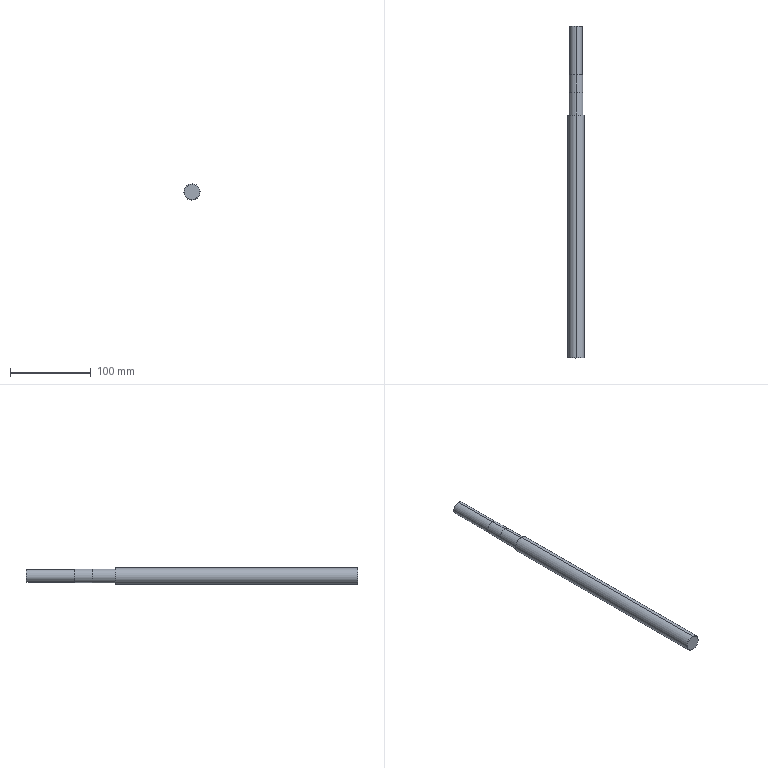Component | SolidWorks | ScrewRod-1 | 1 solid | 29 faces | box 20 x 410 x 20 mm | volume 116845 mm3 | cylinder 13 | cone 8 | plane 8 | commonest cylinder face diameters 5 x5 16 x2 16.7 x2 17 x2 20 x2
build123d program:
from build123d import *

# Parameters (mm, degrees)
SKETCH2_R             = 8.35
BOSS_EXTRUDE1_DEPTH   = 22
SKETCH3_R             = 8
BOSS_EXTRUDE2_DEPTH   = 60
CUT_EXTRUDE1_START    = -5
CUT_EXTRUDE1_DEPTH    = 10
M6_TAPPED_HOLE1_D     = 5
M6_TAPPED_HOLE1_DEPTH = 15
M6_TAPPED_HOLE1_TIP   = 1.502
CHAMFER1_SIZE         = 0.5
CHAMFER2_SIZE         = 0.5


with BuildPart() as part:
    # Sketch1 → Revolve1 (revolve)
    with BuildSketch(Plane.XY, mode=Mode.PRIVATE) as revolve1_sk:
        Polygon((0, 0), (0, 10), (300, 10), (300, 8.5), (328, 8.5), (328, 0), align=None)
    revolve(revolve1_sk.sketch.rotate(Axis((-359.572, 0, 0), (1, 0, 0)), 90), axis=Axis((-359.572, 0, 0), (1, 0, 0)))

    # Sketch2 → Boss-Extrude1 (add)
    with BuildSketch(Plane(origin=(328, 0, 0), x_dir=(0, 0, -1), z_dir=(1, 0, 0))):
        with Locations(Location((0, 0, 0), (0, 0, 180))):
            Circle(SKETCH2_R)
    extrude(amount=BOSS_EXTRUDE1_DEPTH)

    # Sketch3 → Boss-Extrude2 (add)
    with BuildSketch(Plane(origin=(350, 0, 0), x_dir=(0, 0, -1), z_dir=(1, 0, 0))):
        Circle(SKETCH3_R)
    extrude(amount=BOSS_EXTRUDE2_DEPTH)

    # Sketch4 → Cut-Extrude1 (cut)
    with BuildSketch(Plane.XY.offset(CUT_EXTRUDE1_START)):
        with BuildLine():
            Line((387, 2.5), (405, 2.5))
            ThreePointArc((405, 2.5), (407.5, 0), (405, -2.5))
            Line((405, -2.5), (387, -2.5))
            ThreePointArc((387, -2.5), (384.5, 0), (387, 2.5))
        make_face()
    extrude(amount=-CUT_EXTRUDE1_DEPTH, mode=Mode.SUBTRACT)

    # M6 Tapped Hole1
    with Locations(Plane(origin=(410, 0, 0), x_dir=(0, 0, -1), z_dir=(1, 0, 0))):
        with Locations((0, 0)):
            Hole(M6_TAPPED_HOLE1_D / 2, depth=M6_TAPPED_HOLE1_DEPTH)
            with Locations((0, 0, -(M6_TAPPED_HOLE1_DEPTH + M6_TAPPED_HOLE1_TIP / 2))):  # 118° drill point
                Cone(0, M6_TAPPED_HOLE1_D / 2, M6_TAPPED_HOLE1_TIP, mode=Mode.SUBTRACT)

    # Chamfer1
    chamfer1_edges = [part.edges().sort_by_distance(p)[0] for p in [
        (300, 0, -10),
        (0, 0, -10),
    ]]
    chamfer(chamfer1_edges, length=CHAMFER1_SIZE)

    # Chamfer2
    chamfer2_edges = [part.edges().sort_by_distance(p)[0] for p in [
        (410, 0, 8),
    ]]
    chamfer(chamfer2_edges, length=CHAMFER2_SIZE)


solid = part.part

# Placed as in the assembly
solid = solid.moved(Location((-29.507, -82.411, 458), (0, 2.248, 90)))
STEP:
#1=COLOUR_RGB('',0.7922,0.8196,0.9333);
#2=FILL_AREA_STYLE_COLOUR('',#1);
#3=FILL_AREA_STYLE('',(#2));
#4=SURFACE_STYLE_FILL_AREA(#3);
#5=SURFACE_SIDE_STYLE('',(#4));
#6=SURFACE_STYLE_USAGE(.BOTH.,#5);
#7=PRESENTATION_STYLE_ASSIGNMENT((#6));
#8=CARTESIAN_POINT('',(-1.173,12.897,17.736));
#9=VERTEX_POINT('',#8);
#10=CARTESIAN_POINT('',(-1.15,12.897,18.327));
#11=VERTEX_POINT('',#10);
#12=CARTESIAN_POINT('',(-1.162,12.897,18.031));
#13=DIRECTION('',(0.,1.,0.));
#14=DIRECTION('',(-0.03922,0.,-0.9992));
#15=AXIS2_PLACEMENT_3D('',#12,#13,#14);
#16=CIRCLE('',#15,0.2953);
#17=EDGE_CURVE('',#9,#11,#16,.T.);
#18=ORIENTED_EDGE('',*,*,#17,.F.);
#19=CARTESIAN_POINT('',(-1.174,12.878,17.717));
#20=VERTEX_POINT('',#19);
#21=CARTESIAN_POINT('',(-1.173,12.897,17.736));
#22=DIRECTION('',(-0.02773,-0.7071,-0.7066));
#23=VECTOR('',#22,39.37);
#24=LINE('',#21,#23);
#25=EDGE_CURVE('',#9,#20,#24,.T.);
#26=ORIENTED_EDGE('',*,*,#25,.T.);
#27=CARTESIAN_POINT('',(-1.149,12.878,18.346));
#28=VERTEX_POINT('',#27);
#29=CARTESIAN_POINT('',(-1.162,12.878,18.031));
#30=DIRECTION('',(0.,-1.,0.));
#31=DIRECTION('',(-0.03922,0.,-0.9992));
#32=AXIS2_PLACEMENT_3D('',#29,#30,#31);
#33=CIRCLE('',#32,0.315);
#34=EDGE_CURVE('',#28,#20,#33,.T.);
#35=ORIENTED_EDGE('',*,*,#34,.F.);
#36=CARTESIAN_POINT('',(-1.15,12.897,18.327));
#37=DIRECTION('',(0.02773,-0.7071,0.7066));
#38=VECTOR('',#37,39.37);
#39=LINE('',#36,#38);
#40=EDGE_CURVE('',#11,#28,#39,.T.);
#41=ORIENTED_EDGE('',*,*,#40,.F.);
#42=EDGE_LOOP('',(#18,#26,#35,#41));
#43=FACE_OUTER_BOUND('',#42,.T.);
#44=CARTESIAN_POINT('',(-1.162,12.897,18.031));
#45=DIRECTION('',(0.,-1.,0.));
#46=DIRECTION('',(0.03922,0.,0.9992));
#47=AXIS2_PLACEMENT_3D('',#44,#45,#46);
#48=CONICAL_SURFACE('',#47,0.2953,0.7854);
#49=ADVANCED_FACE('',(#43),#48,.T.);
#50=CARTESIAN_POINT('',(-1.176,8.566,17.658));
#51=VERTEX_POINT('',#50);
#52=CARTESIAN_POINT('',(-1.147,8.566,18.405));
#53=VERTEX_POINT('',#52);
#54=CARTESIAN_POINT('',(-1.162,8.566,18.031));
#55=DIRECTION('',(0.,1.,0.));
#56=DIRECTION('',(0.03922,0.,0.9992));
#57=AXIS2_PLACEMENT_3D('',#54,#55,#56);
#58=CIRCLE('',#57,0.374);
#59=EDGE_CURVE('',#51,#53,#58,.T.);
#60=ORIENTED_EDGE('',*,*,#59,.F.);
#61=CARTESIAN_POINT('',(-1.177,8.547,17.638));
#62=VERTEX_POINT('',#61);
#63=CARTESIAN_POINT('',(-1.177,8.547,17.638));
#64=DIRECTION('',(-0.02773,-0.7071,-0.7066));
#65=VECTOR('',#64,39.37);
#66=LINE('',#63,#65);
#67=EDGE_CURVE('',#51,#62,#66,.T.);
#68=ORIENTED_EDGE('',*,*,#67,.T.);
#69=CARTESIAN_POINT('',(-1.146,8.547,18.425));
#70=VERTEX_POINT('',#69);
#71=CARTESIAN_POINT('',(-1.162,8.547,18.031));
#72=DIRECTION('',(0.,-1.,0.));
#73=DIRECTION('',(0.03922,0.,0.9992));
#74=AXIS2_PLACEMENT_3D('',#71,#72,#73);
#75=CIRCLE('',#74,0.3937);
#76=EDGE_CURVE('',#70,#62,#75,.T.);
#77=ORIENTED_EDGE('',*,*,#76,.F.);
#78=CARTESIAN_POINT('',(-1.146,8.547,18.425));
#79=DIRECTION('',(0.02773,-0.7071,0.7066));
#80=VECTOR('',#79,39.37);
#81=LINE('',#78,#80);
#82=EDGE_CURVE('',#53,#70,#81,.T.);
#83=ORIENTED_EDGE('',*,*,#82,.F.);
#84=EDGE_LOOP('',(#60,#68,#77,#83));
#85=FACE_OUTER_BOUND('',#84,.T.);
#86=CARTESIAN_POINT('',(-1.162,8.547,18.031));
#87=DIRECTION('',(0.,-1.,0.));
#88=DIRECTION('',(0.03922,0.,0.9992));
#89=AXIS2_PLACEMENT_3D('',#86,#87,#88);
#90=CONICAL_SURFACE('',#89,0.3937,0.7854);
#91=ADVANCED_FACE('',(#85),#90,.T.);
#92=CARTESIAN_POINT('',(-1.147,-3.245,18.405));
#93=VERTEX_POINT('',#92);
#94=CARTESIAN_POINT('',(-1.176,-3.245,17.658));
#95=VERTEX_POINT('',#94);
#96=CARTESIAN_POINT('',(-1.162,-3.245,18.031));
#97=DIRECTION('',(0.,-1.,0.));
#98=DIRECTION('',(-0.03922,0.,-0.9992));
#99=AXIS2_PLACEMENT_3D('',#96,#97,#98);
#100=CIRCLE('',#99,0.374);
#101=EDGE_CURVE('',#93,#95,#100,.T.);
#102=ORIENTED_EDGE('',*,*,#101,.F.);
#103=CARTESIAN_POINT('',(-1.146,-3.225,18.425));
#104=VERTEX_POINT('',#103);
#105=CARTESIAN_POINT('',(-1.147,-3.245,18.405));
#106=DIRECTION('',(0.02773,0.7071,0.7066));
#107=VECTOR('',#106,39.37);
#108=LINE('',#105,#107);
#109=EDGE_CURVE('',#93,#104,#108,.T.);
#110=ORIENTED_EDGE('',*,*,#109,.T.);
#111=CARTESIAN_POINT('',(-1.177,-3.225,17.638));
#112=VERTEX_POINT('',#111);
#113=CARTESIAN_POINT('',(-1.162,-3.225,18.031));
#114=DIRECTION('',(0.,1.,0.));
#115=DIRECTION('',(-0.03922,0.,-0.9992));
#116=AXIS2_PLACEMENT_3D('',#113,#114,#115);
#117=CIRCLE('',#116,0.3937);
#118=EDGE_CURVE('',#112,#104,#117,.T.);
#119=ORIENTED_EDGE('',*,*,#118,.F.);
#120=CARTESIAN_POINT('',(-1.176,-3.245,17.658));
#121=DIRECTION('',(-0.02773,0.7071,-0.7066));
#122=VECTOR('',#121,39.37);
#123=LINE('',#120,#122);
#124=EDGE_CURVE('',#95,#112,#123,.T.);
#125=ORIENTED_EDGE('',*,*,#124,.F.);
#126=EDGE_LOOP('',(#102,#110,#119,#125));
#127=FACE_OUTER_BOUND('',#126,.T.);
#128=CARTESIAN_POINT('',(-1.162,-3.245,18.031));
#129=DIRECTION('',(0.,1.,0.));
#130=DIRECTION('',(-0.03922,0.,-0.9992));
#131=AXIS2_PLACEMENT_3D('',#128,#129,#130);
#132=CONICAL_SURFACE('',#131,0.374,0.7854);
#133=ADVANCED_FACE('',(#127),#132,.T.);
#134=CARTESIAN_POINT('',(-1.158,12.307,18.13));
#135=VERTEX_POINT('',#134);
#136=CARTESIAN_POINT('',(-1.166,12.307,17.933));
#137=VERTEX_POINT('',#136);
#138=CARTESIAN_POINT('',(-1.162,12.307,18.031));
#139=DIRECTION('',(0.,1.,0.));
#140=DIRECTION('',(-0.03922,0.,-0.9992));
#141=AXIS2_PLACEMENT_3D('',#138,#139,#140);
#142=CIRCLE('',#141,0.09843);
#143=EDGE_CURVE('',#135,#137,#142,.T.);
#144=ORIENTED_EDGE('',*,*,#143,.F.);
#145=CARTESIAN_POINT('',(-1.158,12.897,18.13));
#146=VERTEX_POINT('',#145);
#147=CARTESIAN_POINT('',(-1.158,12.897,18.13));
#148=DIRECTION('',(0.,1.,0.));
#149=VECTOR('',#148,39.37);
#150=LINE('',#147,#149);
#151=EDGE_CURVE('',#135,#146,#150,.T.);
#152=ORIENTED_EDGE('',*,*,#151,.T.);
#153=CARTESIAN_POINT('',(-1.166,12.897,17.933));
#154=VERTEX_POINT('',#153);
#155=CARTESIAN_POINT('',(-1.162,12.897,18.031));
#156=DIRECTION('',(0.,1.,0.));
#157=DIRECTION('',(-0.03922,0.,-0.9992));
#158=AXIS2_PLACEMENT_3D('',#155,#156,#157);
#159=CIRCLE('',#158,0.09843);
#160=EDGE_CURVE('',#146,#154,#159,.T.);
#161=ORIENTED_EDGE('',*,*,#160,.T.);
#162=CARTESIAN_POINT('',(-1.166,12.897,17.933));
#163=DIRECTION('',(0.,1.,0.));
#164=VECTOR('',#163,39.37);
#165=LINE('',#162,#164);
#166=EDGE_CURVE('',#137,#154,#165,.T.);
#167=ORIENTED_EDGE('',*,*,#166,.F.);
#168=EDGE_LOOP('',(#144,#152,#161,#167));
#169=FACE_OUTER_BOUND('',#168,.T.);
#170=CARTESIAN_POINT('',(-1.162,12.897,18.031));
#171=DIRECTION('',(0.,1.,0.));
#172=DIRECTION('',(-0.03922,0.,-0.9992));
#173=AXIS2_PLACEMENT_3D('',#170,#171,#172);
#174=CYLINDRICAL_SURFACE('',#173,0.09843);
#175=ADVANCED_FACE('',(#169),#174,.F.);
#176=CARTESIAN_POINT('',(-1.162,12.248,18.031));
#177=VERTEX_POINT('',#176);
#178=CARTESIAN_POINT('',(-1.166,12.307,17.933));
#179=DIRECTION('',(-0.03362,0.515,-0.8565));
#180=VECTOR('',#179,39.37);
#181=LINE('',#178,#180);
#182=EDGE_CURVE('',#177,#137,#181,.T.);
#183=ORIENTED_EDGE('',*,*,#182,.F.);
#184=CARTESIAN_POINT('',(-1.158,12.307,18.13));
#185=DIRECTION('',(0.03362,0.515,0.8565));
#186=VECTOR('',#185,39.37);
#187=LINE('',#184,#186);
#188=EDGE_CURVE('',#177,#135,#187,.T.);
#189=ORIENTED_EDGE('',*,*,#188,.T.);
#190=ORIENTED_EDGE('',*,*,#143,.T.);
#191=EDGE_LOOP('',(#183,#189,#190));
#192=FACE_OUTER_BOUND('',#191,.T.);
#193=CARTESIAN_POINT('',(-1.162,12.307,18.031));
#194=DIRECTION('',(0.,1.,0.));
#195=DIRECTION('',(-0.03922,0.,-0.9992));
#196=AXIS2_PLACEMENT_3D('',#193,#194,#195);
#197=CONICAL_SURFACE('',#196,0.09843,1.03);
#198=ADVANCED_FACE('',(#192),#197,.F.);
#199=CARTESIAN_POINT('',(-1.174,12.799,17.717));
#200=VERTEX_POINT('',#199);
#201=CARTESIAN_POINT('',(-1.272,12.7,17.736));
#202=VERTEX_POINT('',#201);
#203=CARTESIAN_POINT('',(-1.174,12.799,17.717));
#204=CARTESIAN_POINT('',(-1.18,12.799,17.717));
#205=CARTESIAN_POINT('',(-1.187,12.798,17.717));
#206=CARTESIAN_POINT('',(-1.2,12.796,17.719));
#207=CARTESIAN_POINT('',(-1.206,12.794,17.72));
#208=CARTESIAN_POINT('',(-1.218,12.789,17.721));
#209=CARTESIAN_POINT('',(-1.223,12.786,17.723));
#210=CARTESIAN_POINT('',(-1.234,12.779,17.725));
#211=CARTESIAN_POINT('',(-1.239,12.774,17.726));
#212=CARTESIAN_POINT('',(-1.248,12.765,17.728));
#213=CARTESIAN_POINT('',(-1.252,12.76,17.73));
#214=CARTESIAN_POINT('',(-1.259,12.75,17.732));
#215=CARTESIAN_POINT('',(-1.262,12.744,17.733));
#216=CARTESIAN_POINT('',(-1.267,12.732,17.735));
#217=CARTESIAN_POINT('',(-1.269,12.726,17.735));
#218=CARTESIAN_POINT('',(-1.271,12.713,17.736));
#219=CARTESIAN_POINT('',(-1.272,12.707,17.736));
#220=CARTESIAN_POINT('',(-1.272,12.7,17.736));
#221=B_SPLINE_CURVE_WITH_KNOTS('',3,(#203,#204,#205,#206,#207,#208,#209,#210,#211,#212,#213,#214,#215,#216,#217,#218,#219,#220),.UNSPECIFIED.,.F.,.F.,(4,2,2,2,2,2,2,2,4),(0.003934,0.004425,0.004916,0.005407,0.005898,0.006389,0.006881,0.007372,0.007863),.UNSPECIFIED.);
#222=EDGE_CURVE('',#200,#202,#221,.T.);
#223=ORIENTED_EDGE('',*,*,#222,.F.);
#224=CARTESIAN_POINT('',(-1.169,12.799,17.835));
#225=VERTEX_POINT('',#224);
#226=CARTESIAN_POINT('',(-1.185,12.799,17.441));
#227=DIRECTION('',(0.03922,0.,0.9992));
#228=VECTOR('',#227,39.37);
#229=LINE('',#226,#228);
#230=EDGE_CURVE('',#200,#225,#229,.T.);
#231=ORIENTED_EDGE('',*,*,#230,.T.);
#232=CARTESIAN_POINT('',(-1.268,12.7,17.839));
#233=VERTEX_POINT('',#232);
#234=CARTESIAN_POINT('',(-1.169,12.7,17.835));
#235=DIRECTION('',(0.03922,0.,0.9992));
#236=DIRECTION('',(0.,1.,0.));
#237=AXIS2_PLACEMENT_3D('',#234,#235,#236);
#238=CIRCLE('',#237,0.09843);
#239=EDGE_CURVE('',#225,#233,#238,.T.);
#240=ORIENTED_EDGE('',*,*,#239,.T.);
#241=CARTESIAN_POINT('',(-1.283,12.7,17.445));
#242=DIRECTION('',(0.03922,0.,0.9992));
#243=VECTOR('',#242,39.37);
#244=LINE('',#241,#243);
#245=EDGE_CURVE('',#202,#233,#244,.T.);
#246=ORIENTED_EDGE('',*,*,#245,.F.);
#247=EDGE_LOOP('',(#223,#231,#240,#246));
#248=FACE_OUTER_BOUND('',#247,.T.);
#249=CARTESIAN_POINT('',(-1.185,12.7,17.441));
#250=DIRECTION('',(0.03922,0.,0.9992));
#251=DIRECTION('',(0.,1.,0.));
#252=AXIS2_PLACEMENT_3D('',#249,#250,#251);
#253=CYLINDRICAL_SURFACE('',#252,0.09843);
#254=ADVANCED_FACE('',(#248),#253,.F.);
#255=ORIENTED_EDGE('',*,*,#34,.T.);
#256=CARTESIAN_POINT('',(-1.174,12.897,17.717));
#257=DIRECTION('',(0.,-1.,0.));
#258=VECTOR('',#257,39.37);
#259=LINE('',#256,#258);
#260=EDGE_CURVE('',#20,#200,#259,.T.);
#261=ORIENTED_EDGE('',*,*,#260,.T.);
#262=ORIENTED_EDGE('',*,*,#222,.T.);
#263=CARTESIAN_POINT('',(-1.272,11.992,17.736));
#264=VERTEX_POINT('',#263);
#265=CARTESIAN_POINT('',(-1.272,12.897,17.736));
#266=DIRECTION('',(0.,-1.,0.));
#267=VECTOR('',#266,39.37);
#268=LINE('',#265,#267);
#269=EDGE_CURVE('',#202,#264,#268,.T.);
#270=ORIENTED_EDGE('',*,*,#269,.T.);
#271=CARTESIAN_POINT('',(-1.174,11.893,17.717));
#272=VERTEX_POINT('',#271);
#273=CARTESIAN_POINT('',(-1.272,11.992,17.736));
#274=CARTESIAN_POINT('',(-1.272,11.985,17.736));
#275=CARTESIAN_POINT('',(-1.271,11.979,17.736));
#276=CARTESIAN_POINT('',(-1.269,11.966,17.735));
#277=CARTESIAN_POINT('',(-1.267,11.96,17.735));
#278=CARTESIAN_POINT('',(-1.262,11.948,17.733));
#279=CARTESIAN_POINT('',(-1.259,11.942,17.732));
#280=CARTESIAN_POINT('',(-1.252,11.932,17.73));
#281=CARTESIAN_POINT('',(-1.248,11.927,17.728));
#282=CARTESIAN_POINT('',(-1.234,11.913,17.725));
#283=CARTESIAN_POINT('',(-1.223,11.906,17.722));
#284=CARTESIAN_POINT('',(-1.206,11.898,17.72));
#285=CARTESIAN_POINT('',(-1.2,11.896,17.719));
#286=CARTESIAN_POINT('',(-1.187,11.894,17.717));
#287=CARTESIAN_POINT('',(-1.18,11.893,17.717));
#288=CARTESIAN_POINT('',(-1.174,11.893,17.717));
#289=B_SPLINE_CURVE_WITH_KNOTS('',3,(#273,#274,#275,#276,#277,#278,#279,#280,#281,#282,#283,#284,#285,#286,#287,#288),.UNSPECIFIED.,.F.,.F.,(4,2,2,2,2,2,2,4),(0.,0.0004917,0.0009835,0.001475,0.001967,0.00295,0.003442,0.003934),.UNSPECIFIED.);
#290=EDGE_CURVE('',#264,#272,#289,.T.);
#291=ORIENTED_EDGE('',*,*,#290,.T.);
#292=CARTESIAN_POINT('',(-1.174,10.535,17.717));
#293=VERTEX_POINT('',#292);
#294=CARTESIAN_POINT('',(-1.174,12.897,17.717));
#295=DIRECTION('',(0.,-1.,0.));
#296=VECTOR('',#295,39.37);
#297=LINE('',#294,#296);
#298=EDGE_CURVE('',#272,#293,#297,.T.);
#299=ORIENTED_EDGE('',*,*,#298,.T.);
#300=CARTESIAN_POINT('',(-1.149,10.535,18.346));
#301=VERTEX_POINT('',#300);
#302=CARTESIAN_POINT('',(-1.162,10.535,18.031));
#303=DIRECTION('',(0.,1.,0.));
#304=DIRECTION('',(-0.03922,0.,-0.9992));
#305=AXIS2_PLACEMENT_3D('',#302,#303,#304);
#306=CIRCLE('',#305,0.315);
#307=EDGE_CURVE('',#293,#301,#306,.T.);
#308=ORIENTED_EDGE('',*,*,#307,.T.);
#309=CARTESIAN_POINT('',(-1.149,12.897,18.346));
#310=DIRECTION('',(0.,-1.,0.));
#311=VECTOR('',#310,39.37);
#312=LINE('',#309,#311);
#313=EDGE_CURVE('',#28,#301,#312,.T.);
#314=ORIENTED_EDGE('',*,*,#313,.F.);
#315=EDGE_LOOP('',(#255,#261,#262,#270,#291,#299,#308,#314));
#316=FACE_OUTER_BOUND('',#315,.T.);
#317=CARTESIAN_POINT('',(-1.162,12.897,18.031));
#318=DIRECTION('',(0.,-1.,0.));
#319=DIRECTION('',(0.03922,0.,0.9992));
#320=AXIS2_PLACEMENT_3D('',#317,#318,#319);
#321=CYLINDRICAL_SURFACE('',#320,0.315);
#322=ADVANCED_FACE('',(#316),#321,.T.);
#323=CARTESIAN_POINT('',(-1.175,10.535,17.703));
#324=VERTEX_POINT('',#323);
#325=CARTESIAN_POINT('',(-1.149,10.535,18.36));
#326=VERTEX_POINT('',#325);
#327=CARTESIAN_POINT('',(-1.162,10.535,18.031));
#328=DIRECTION('',(0.,1.,0.));
#329=DIRECTION('',(-0.03922,0.,-0.9992));
#330=AXIS2_PLACEMENT_3D('',#327,#328,#329);
#331=CIRCLE('',#330,0.3287);
#332=EDGE_CURVE('',#324,#326,#331,.T.);
#333=ORIENTED_EDGE('',*,*,#332,.F.);
#334=CARTESIAN_POINT('',(-1.175,9.669,17.703));
#335=VERTEX_POINT('',#334);
#336=CARTESIAN_POINT('',(-1.175,10.535,17.703));
#337=DIRECTION('',(0.,-1.,0.));
#338=VECTOR('',#337,39.37);
#339=LINE('',#336,#338);
#340=EDGE_CURVE('',#324,#335,#339,.T.);
#341=ORIENTED_EDGE('',*,*,#340,.T.);
#342=CARTESIAN_POINT('',(-1.149,9.669,18.36));
#343=VERTEX_POINT('',#342);
#344=CARTESIAN_POINT('',(-1.162,9.669,18.031));
#345=DIRECTION('',(0.,1.,0.));
#346=DIRECTION('',(0.03922,0.,0.9992));
#347=AXIS2_PLACEMENT_3D('',#344,#345,#346);
#348=CIRCLE('',#347,0.3287);
#349=EDGE_CURVE('',#335,#343,#348,.T.);
#350=ORIENTED_EDGE('',*,*,#349,.T.);
#351=CARTESIAN_POINT('',(-1.149,10.535,18.36));
#352=DIRECTION('',(0.,-1.,0.));
#353=VECTOR('',#352,39.37);
#354=LINE('',#351,#353);
#355=EDGE_CURVE('',#326,#343,#354,.T.);
#356=ORIENTED_EDGE('',*,*,#355,.F.);
#357=EDGE_LOOP('',(#333,#341,#350,#356));
#358=FACE_OUTER_BOUND('',#357,.T.);
#359=CARTESIAN_POINT('',(-1.162,10.535,18.031));
#360=DIRECTION('',(0.,-1.,0.));
#361=DIRECTION('',(0.03922,0.,0.9992));
#362=AXIS2_PLACEMENT_3D('',#359,#360,#361);
#363=CYLINDRICAL_SURFACE('',#362,0.3287);
#364=ADVANCED_FACE('',(#358),#363,.T.);
#365=CARTESIAN_POINT('',(-1.149,9.669,18.366));
#366=VERTEX_POINT('',#365);
#367=CARTESIAN_POINT('',(-1.175,9.669,17.697));
#368=VERTEX_POINT('',#367);
#369=CARTESIAN_POINT('',(-1.162,9.669,18.031));
#370=DIRECTION('',(0.,-1.,0.));
#371=DIRECTION('',(0.03922,0.,0.9992));
#372=AXIS2_PLACEMENT_3D('',#369,#370,#371);
#373=CIRCLE('',#372,0.3346);
#374=EDGE_CURVE('',#366,#368,#373,.T.);
#375=ORIENTED_EDGE('',*,*,#374,.T.);
#376=CARTESIAN_POINT('',(-1.175,8.566,17.697));
#377=VERTEX_POINT('',#376);
#378=CARTESIAN_POINT('',(-1.175,-17.401,17.697));
#379=DIRECTION('',(0.,-1.,0.));
#380=VECTOR('',#379,39.37);
#381=LINE('',#378,#380);
#382=EDGE_CURVE('',#368,#377,#381,.T.);
#383=ORIENTED_EDGE('',*,*,#382,.T.);
#384=CARTESIAN_POINT('',(-1.149,8.566,18.366));
#385=VERTEX_POINT('',#384);
#386=CARTESIAN_POINT('',(-1.162,8.566,18.031));
#387=DIRECTION('',(0.,-1.,0.));
#388=DIRECTION('',(0.03922,0.,0.9992));
#389=AXIS2_PLACEMENT_3D('',#386,#387,#388);
#390=CIRCLE('',#389,0.3346);
#391=EDGE_CURVE('',#385,#377,#390,.T.);
#392=ORIENTED_EDGE('',*,*,#391,.F.);
#393=CARTESIAN_POINT('',(-1.149,-17.401,18.366));
#394=DIRECTION('',(0.,-1.,0.));
#395=VECTOR('',#394,39.37);
#396=LINE('',#393,#395);
#397=EDGE_CURVE('',#366,#385,#396,.T.);
#398=ORIENTED_EDGE('',*,*,#397,.F.);
#399=EDGE_LOOP('',(#375,#383,#392,#398));
#400=FACE_OUTER_BOUND('',#399,.T.);
#401=CARTESIAN_POINT('',(-1.162,-17.401,18.031));
#402=DIRECTION('',(0.,-1.,0.));
#403=DIRECTION('',(0.03922,0.,0.9992));
#404=AXIS2_PLACEMENT_3D('',#401,#402,#403);
#405=CYLINDRICAL_SURFACE('',#404,0.3346);
#406=ADVANCED_FACE('',(#400),#405,.T.);
#407=ORIENTED_EDGE('',*,*,#76,.T.);
#408=CARTESIAN_POINT('',(-1.177,-17.401,17.638));
#409=DIRECTION('',(0.,-1.,0.));
#410=VECTOR('',#409,39.37);
#411=LINE('',#408,#410);
#412=EDGE_CURVE('',#62,#112,#411,.T.);
#413=ORIENTED_EDGE('',*,*,#412,.T.);
#414=ORIENTED_EDGE('',*,*,#118,.T.);
#415=CARTESIAN_POINT('',(-1.146,-17.401,18.425));
#416=DIRECTION('',(0.,-1.,0.));
#417=VECTOR('',#416,39.37);
#418=LINE('',#415,#417);
#419=EDGE_CURVE('',#70,#104,#418,.T.);
#420=ORIENTED_EDGE('',*,*,#419,.F.);
#421=EDGE_LOOP('',(#407,#413,#414,#420));
#422=FACE_OUTER_BOUND('',#421,.T.);
#423=CARTESIAN_POINT('',(-1.162,-17.401,18.031));
#424=DIRECTION('',(0.,-1.,0.));
#425=DIRECTION('',(0.03922,0.,0.9992));
#426=AXIS2_PLACEMENT_3D('',#423,#424,#425);
#427=CYLINDRICAL_SURFACE('',#426,0.3937);
#428=ADVANCED_FACE('',(#422),#427,.T.);
#429=CARTESIAN_POINT('',(-1.162,-3.245,18.031));
#430=DIRECTION('',(0.,-1.,0.));
#431=DIRECTION('',(-0.03922,0.,-0.9992));
#432=AXIS2_PLACEMENT_3D('',#429,#430,#431);
#433=CIRCLE('',#432,0.374);
#434=EDGE_CURVE('',#95,#93,#433,.T.);
#435=ORIENTED_EDGE('',*,*,#434,.T.);
#436=ORIENTED_EDGE('',*,*,#101,.T.);
#437=EDGE_LOOP('',(#435,#436));
#438=FACE_OUTER_BOUND('',#437,.T.);
#439=CARTESIAN_POINT('',(-1.162,-3.245,18.031));
#440=DIRECTION('',(0.,1.,0.));
#441=DIRECTION('',(-0.03922,0.,-0.9992));
#442=AXIS2_PLACEMENT_3D('',#439,#440,#441);
#443=PLANE('',#442);
#444=ADVANCED_FACE('',(#438),#443,.F.);
#445=ORIENTED_EDGE('',*,*,#412,.F.);
#446=CARTESIAN_POINT('',(-1.162,8.547,18.031));
#447=DIRECTION('',(0.,-1.,0.));
#448=DIRECTION('',(0.03922,0.,0.9992));
#449=AXIS2_PLACEMENT_3D('',#446,#447,#448);
#450=CIRCLE('',#449,0.3937);
#451=EDGE_CURVE('',#62,#70,#450,.T.);
#452=ORIENTED_EDGE('',*,*,#451,.T.);
#453=ORIENTED_EDGE('',*,*,#419,.T.);
#454=CARTESIAN_POINT('',(-1.162,-3.225,18.031));
#455=DIRECTION('',(0.,1.,0.));
#456=DIRECTION('',(-0.03922,0.,-0.9992));
#457=AXIS2_PLACEMENT_3D('',#454,#455,#456);
#458=CIRCLE('',#457,0.3937);
#459=EDGE_CURVE('',#104,#112,#458,.T.);
#460=ORIENTED_EDGE('',*,*,#459,.T.);
#461=EDGE_LOOP('',(#445,#452,#453,#460));
#462=FACE_OUTER_BOUND('',#461,.T.);
#463=CARTESIAN_POINT('',(-1.162,-17.401,18.031));
#464=DIRECTION('',(0.,-1.,0.));
#465=DIRECTION('',(0.03922,0.,0.9992));
#466=AXIS2_PLACEMENT_3D('',#463,#464,#465);
#467=CYLINDRICAL_SURFACE('',#466,0.3937);
#468=ADVANCED_FACE('',(#462),#467,.T.);
#469=CARTESIAN_POINT('',(-1.162,8.566,18.031));
#470=DIRECTION('',(0.,1.,0.));
#471=DIRECTION('',(0.03922,0.,0.9992));
#472=AXIS2_PLACEMENT_3D('',#469,#470,#471);
#473=CIRCLE('',#472,0.374);
#474=EDGE_CURVE('',#53,#51,#473,.T.);
#475=ORIENTED_EDGE('',*,*,#474,.T.);
#476=ORIENTED_EDGE('',*,*,#59,.T.);
#477=EDGE_LOOP('',(#475,#476));
#478=FACE_OUTER_BOUND('',#477,.T.);
#479=ORIENTED_EDGE('',*,*,#391,.T.);
#480=CARTESIAN_POINT('',(-1.162,8.566,18.031));
#481=DIRECTION('',(0.,-1.,0.));
#482=DIRECTION('',(0.03922,0.,0.9992));
#483=AXIS2_PLACEMENT_3D('',#480,#481,#482);
#484=CIRCLE('',#483,0.3346);
#485=EDGE_CURVE('',#377,#385,#484,.T.);
#486=ORIENTED_EDGE('',*,*,#485,.T.);
#487=EDGE_LOOP('',(#479,#486));
#488=FACE_BOUND('',#487,.T.);
#489=CARTESIAN_POINT('',(-1.555,8.566,18.047));
#490=DIRECTION('',(0.,-1.,0.));
#491=DIRECTION('',(0.03922,0.,0.9992));
#492=AXIS2_PLACEMENT_3D('',#489,#490,#491);
#493=PLANE('',#492);
#494=ADVANCED_FACE('',(#478,#488),#493,.F.);
#495=ORIENTED_EDGE('',*,*,#382,.F.);
#496=CARTESIAN_POINT('',(-1.162,9.669,18.031));
#497=DIRECTION('',(0.,-1.,0.));
#498=DIRECTION('',(0.03922,0.,0.9992));
#499=AXIS2_PLACEMENT_3D('',#496,#497,#498);
#500=CIRCLE('',#499,0.3346);
#501=EDGE_CURVE('',#368,#366,#500,.T.);
#502=ORIENTED_EDGE('',*,*,#501,.T.);
#503=ORIENTED_EDGE('',*,*,#397,.T.);
#504=ORIENTED_EDGE('',*,*,#485,.F.);
#505=EDGE_LOOP('',(#495,#502,#503,#504));
#506=FACE_OUTER_BOUND('',#505,.T.);
#507=CARTESIAN_POINT('',(-1.162,-17.401,18.031));
#508=DIRECTION('',(0.,-1.,0.));
#509=DIRECTION('',(0.03922,0.,0.9992));
#510=AXIS2_PLACEMENT_3D('',#507,#508,#509);
#511=CYLINDRICAL_SURFACE('',#510,0.3346);
#512=ADVANCED_FACE('',(#506),#511,.T.);
#513=CARTESIAN_POINT('',(-1.162,9.669,18.031));
#514=DIRECTION('',(0.,1.,0.));
#515=DIRECTION('',(0.03922,0.,0.9992));
#516=AXIS2_PLACEMENT_3D('',#513,#514,#515);
#517=CIRCLE('',#516,0.3287);
#518=EDGE_CURVE('',#343,#335,#517,.T.);
#519=ORIENTED_EDGE('',*,*,#518,.F.);
#520=ORIENTED_EDGE('',*,*,#349,.F.);
#521=EDGE_LOOP('',(#519,#520));
#522=FACE_BOUND('',#521,.T.);
#523=ORIENTED_EDGE('',*,*,#374,.F.);
#524=ORIENTED_EDGE('',*,*,#501,.F.);
#525=EDGE_LOOP('',(#523,#524));
#526=FACE_OUTER_BOUND('',#525,.T.);
#527=CARTESIAN_POINT('',(-1.496,9.669,18.045));
#528=DIRECTION('',(0.,-1.,0.));
#529=DIRECTION('',(0.03922,0.,0.9992));
#530=AXIS2_PLACEMENT_3D('',#527,#528,#529);
#531=PLANE('',#530);
#532=ADVANCED_FACE('',(#522,#526),#531,.F.);
#533=ORIENTED_EDGE('',*,*,#340,.F.);
#534=CARTESIAN_POINT('',(-1.162,10.535,18.031));
#535=DIRECTION('',(0.,1.,0.));
#536=DIRECTION('',(-0.03922,0.,-0.9992));
#537=AXIS2_PLACEMENT_3D('',#534,#535,#536);
#538=CIRCLE('',#537,0.3287);
#539=EDGE_CURVE('',#326,#324,#538,.T.);
#540=ORIENTED_EDGE('',*,*,#539,.F.);
#541=ORIENTED_EDGE('',*,*,#355,.T.);
#542=ORIENTED_EDGE('',*,*,#518,.T.);
#543=EDGE_LOOP('',(#533,#540,#541,#542));
#544=FACE_OUTER_BOUND('',#543,.T.);
#545=CARTESIAN_POINT('',(-1.162,10.535,18.031));
#546=DIRECTION('',(0.,-1.,0.));
#547=DIRECTION('',(0.03922,0.,0.9992));
#548=AXIS2_PLACEMENT_3D('',#545,#546,#547);
#549=CYLINDRICAL_SURFACE('',#548,0.3287);
#550=ADVANCED_FACE('',(#544),#549,.T.);
#551=CARTESIAN_POINT('',(-1.162,10.535,18.031));
#552=DIRECTION('',(0.,1.,0.));
#553=DIRECTION('',(-0.03922,0.,-0.9992));
#554=AXIS2_PLACEMENT_3D('',#551,#552,#553);
#555=CIRCLE('',#554,0.315);
#556=EDGE_CURVE('',#301,#293,#555,.T.);
#557=ORIENTED_EDGE('',*,*,#556,.F.);
#558=ORIENTED_EDGE('',*,*,#307,.F.);
#559=EDGE_LOOP('',(#557,#558));
#560=FACE_BOUND('',#559,.T.);
#561=ORIENTED_EDGE('',*,*,#539,.T.);
#562=ORIENTED_EDGE('',*,*,#332,.T.);
#563=EDGE_LOOP('',(#561,#562));
#564=FACE_OUTER_BOUND('',#563,.T.);
#565=CARTESIAN_POINT('',(-1.162,10.535,18.031));
#566=DIRECTION('',(0.,1.,0.));
#567=DIRECTION('',(-0.03922,0.,-0.9992));
#568=AXIS2_PLACEMENT_3D('',#565,#566,#567);
#569=PLANE('',#568);
#570=ADVANCED_FACE('',(#560,#564),#569,.T.);
#571=ORIENTED_EDGE('',*,*,#260,.F.);
#572=CARTESIAN_POINT('',(-1.162,12.878,18.031));
#573=DIRECTION('',(0.,-1.,0.));
#574=DIRECTION('',(-0.03922,0.,-0.9992));
#575=AXIS2_PLACEMENT_3D('',#572,#573,#574);
#576=CIRCLE('',#575,0.315);
#577=EDGE_CURVE('',#20,#28,#576,.T.);
#578=ORIENTED_EDGE('',*,*,#577,.T.);
#579=ORIENTED_EDGE('',*,*,#313,.T.);
#580=ORIENTED_EDGE('',*,*,#556,.T.);
#581=ORIENTED_EDGE('',*,*,#298,.F.);
#582=CARTESIAN_POINT('',(-1.075,11.992,17.729));
#583=VERTEX_POINT('',#582);
#584=CARTESIAN_POINT('',(-1.174,11.893,17.717));
#585=CARTESIAN_POINT('',(-1.168,11.893,17.717));
#586=CARTESIAN_POINT('',(-1.161,11.894,17.716));
#587=CARTESIAN_POINT('',(-1.148,11.896,17.717));
#588=CARTESIAN_POINT('',(-1.142,11.898,17.717));
#589=CARTESIAN_POINT('',(-1.13,11.903,17.718));
#590=CARTESIAN_POINT('',(-1.124,11.906,17.719));
#591=CARTESIAN_POINT('',(-1.114,11.913,17.72));
#592=CARTESIAN_POINT('',(-1.109,11.918,17.721));
#593=CARTESIAN_POINT('',(-1.1,11.927,17.723));
#594=CARTESIAN_POINT('',(-1.096,11.932,17.724));
#595=CARTESIAN_POINT('',(-1.088,11.942,17.725));
#596=CARTESIAN_POINT('',(-1.085,11.948,17.726));
#597=CARTESIAN_POINT('',(-1.08,11.96,17.727));
#598=CARTESIAN_POINT('',(-1.078,11.966,17.728));
#599=CARTESIAN_POINT('',(-1.076,11.979,17.728));
#600=CARTESIAN_POINT('',(-1.075,11.985,17.729));
#601=CARTESIAN_POINT('',(-1.075,11.992,17.729));
#602=B_SPLINE_CURVE_WITH_KNOTS('',3,(#584,#585,#586,#587,#588,#589,#590,#591,#592,#593,#594,#595,#596,#597,#598,#599,#600,#601),.UNSPECIFIED.,.F.,.F.,(4,2,2,2,2,2,2,2,4),(0.003934,0.004425,0.004916,0.005407,0.005898,0.006389,0.006881,0.007372,0.007863),.UNSPECIFIED.);
#603=EDGE_CURVE('',#272,#583,#602,.T.);
#604=ORIENTED_EDGE('',*,*,#603,.T.);
#605=CARTESIAN_POINT('',(-1.075,12.7,17.729));
#606=VERTEX_POINT('',#605);
#607=CARTESIAN_POINT('',(-1.075,12.897,17.729));
#608=DIRECTION('',(0.,1.,0.));
#609=VECTOR('',#608,39.37);
#610=LINE('',#607,#609);
#611=EDGE_CURVE('',#583,#606,#610,.T.);
#612=ORIENTED_EDGE('',*,*,#611,.T.);
#613=CARTESIAN_POINT('',(-1.075,12.7,17.729));
#614=CARTESIAN_POINT('',(-1.075,12.707,17.729));
#615=CARTESIAN_POINT('',(-1.076,12.713,17.728));
#616=CARTESIAN_POINT('',(-1.078,12.726,17.728));
#617=CARTESIAN_POINT('',(-1.08,12.732,17.727));
#618=CARTESIAN_POINT('',(-1.085,12.744,17.726));
#619=CARTESIAN_POINT('',(-1.088,12.75,17.725));
#620=CARTESIAN_POINT('',(-1.095,12.76,17.724));
#621=CARTESIAN_POINT('',(-1.1,12.765,17.723));
#622=CARTESIAN_POINT('',(-1.113,12.779,17.72));
#623=CARTESIAN_POINT('',(-1.124,12.786,17.719));
#624=CARTESIAN_POINT('',(-1.142,12.794,17.717));
#625=CARTESIAN_POINT('',(-1.148,12.796,17.717));
#626=CARTESIAN_POINT('',(-1.161,12.798,17.716));
#627=CARTESIAN_POINT('',(-1.168,12.799,17.717));
#628=CARTESIAN_POINT('',(-1.174,12.799,17.717));
#629=B_SPLINE_CURVE_WITH_KNOTS('',3,(#613,#614,#615,#616,#617,#618,#619,#620,#621,#622,#623,#624,#625,#626,#627,#628),.UNSPECIFIED.,.F.,.F.,(4,2,2,2,2,2,2,4),(0.,0.0004917,0.0009835,0.001475,0.001967,0.00295,0.003442,0.003934),.UNSPECIFIED.);
#630=EDGE_CURVE('',#606,#200,#629,.T.);
#631=ORIENTED_EDGE('',*,*,#630,.T.);
#632=EDGE_LOOP('',(#571,#578,#579,#580,#581,#604,#612,#631));
#633=FACE_OUTER_BOUND('',#632,.T.);
#634=CARTESIAN_POINT('',(-1.162,12.897,18.031));
#635=DIRECTION('',(0.,-1.,0.));
#636=DIRECTION('',(0.03922,0.,0.9992));
#637=AXIS2_PLACEMENT_3D('',#634,#635,#636);
#638=CYLINDRICAL_SURFACE('',#637,0.315);
#639=ADVANCED_FACE('',(#633),#638,.T.);
#640=CARTESIAN_POINT('',(-1.162,12.897,18.031));
#641=DIRECTION('',(0.,1.,0.));
#642=DIRECTION('',(-0.03922,0.,-0.9992));
#643=AXIS2_PLACEMENT_3D('',#640,#641,#642);
#644=CIRCLE('',#643,0.2953);
#645=EDGE_CURVE('',#11,#9,#644,.T.);
#646=ORIENTED_EDGE('',*,*,#645,.T.);
#647=ORIENTED_EDGE('',*,*,#17,.T.);
#648=EDGE_LOOP('',(#646,#647));
#649=FACE_OUTER_BOUND('',#648,.T.);
#650=CARTESIAN_POINT('',(-1.162,12.897,18.031));
#651=DIRECTION('',(0.,1.,0.));
#652=DIRECTION('',(-0.03922,0.,-0.9992));
#653=AXIS2_PLACEMENT_3D('',#650,#651,#652);
#654=CIRCLE('',#653,0.09843);
#655=EDGE_CURVE('',#154,#146,#654,.T.);
#656=ORIENTED_EDGE('',*,*,#655,.F.);
#657=ORIENTED_EDGE('',*,*,#160,.F.);
#658=EDGE_LOOP('',(#656,#657));
#659=FACE_BOUND('',#658,.T.);
#660=CARTESIAN_POINT('',(-1.162,12.897,18.031));
#661=DIRECTION('',(0.,1.,0.));
#662=DIRECTION('',(-0.03922,0.,-0.9992));
#663=AXIS2_PLACEMENT_3D('',#660,#661,#662);
#664=PLANE('',#663);
#665=ADVANCED_FACE('',(#649,#659),#664,.T.);
#666=CARTESIAN_POINT('',(-1.268,11.992,17.839));
#667=VERTEX_POINT('',#666);
#668=CARTESIAN_POINT('',(-1.283,11.992,17.445));
#669=DIRECTION('',(0.03922,0.,0.9992));
#670=VECTOR('',#669,39.37);
#671=LINE('',#668,#670);
#672=EDGE_CURVE('',#264,#667,#671,.T.);
#673=ORIENTED_EDGE('',*,*,#672,.T.);
#674=CARTESIAN_POINT('',(-1.071,11.992,17.831));
#675=VERTEX_POINT('',#674);
#676=CARTESIAN_POINT('',(-1.169,11.992,17.835));
#677=DIRECTION('',(0.03922,0.,0.9992));
#678=DIRECTION('',(0.,1.,0.));
#679=AXIS2_PLACEMENT_3D('',#676,#677,#678);
#680=CIRCLE('',#679,0.09843);
#681=EDGE_CURVE('',#667,#675,#680,.T.);
#682=ORIENTED_EDGE('',*,*,#681,.T.);
#683=CARTESIAN_POINT('',(-1.086,11.992,17.438));
#684=DIRECTION('',(0.03922,0.,0.9992));
#685=VECTOR('',#684,39.37);
#686=LINE('',#683,#685);
#687=EDGE_CURVE('',#583,#675,#686,.T.);
#688=ORIENTED_EDGE('',*,*,#687,.F.);
#689=ORIENTED_EDGE('',*,*,#603,.F.);
#690=ORIENTED_EDGE('',*,*,#290,.F.);
#691=EDGE_LOOP('',(#673,#682,#688,#689,#690));
#692=FACE_OUTER_BOUND('',#691,.T.);
#693=CARTESIAN_POINT('',(-1.185,11.992,17.441));
#694=DIRECTION('',(0.03922,0.,0.9992));
#695=DIRECTION('',(0.,1.,0.));
#696=AXIS2_PLACEMENT_3D('',#693,#694,#695);
#697=CYLINDRICAL_SURFACE('',#696,0.09843);
#698=ADVANCED_FACE('',(#692),#697,.F.);
#699=ORIENTED_EDGE('',*,*,#245,.T.);
#700=CARTESIAN_POINT('',(-1.268,11.992,17.839));
#701=DIRECTION('',(0.,-1.,-0.));
#702=VECTOR('',#701,39.37);
#703=LINE('',#700,#702);
#704=EDGE_CURVE('',#233,#667,#703,.T.);
#705=ORIENTED_EDGE('',*,*,#704,.T.);
#706=ORIENTED_EDGE('',*,*,#672,.F.);
#707=ORIENTED_EDGE('',*,*,#269,.F.);
#708=EDGE_LOOP('',(#699,#705,#706,#707));
#709=FACE_OUTER_BOUND('',#708,.T.);
#710=CARTESIAN_POINT('',(-1.283,11.992,17.445));
#711=DIRECTION('',(-0.9992,-0.,0.03922));
#712=DIRECTION('',(0.,-1.,-0.));
#713=AXIS2_PLACEMENT_3D('',#710,#711,#712);
#714=PLANE('',#713);
#715=ADVANCED_FACE('',(#709),#714,.F.);
#716=ORIENTED_EDGE('',*,*,#230,.F.);
#717=ORIENTED_EDGE('',*,*,#630,.F.);
#718=CARTESIAN_POINT('',(-1.071,12.7,17.831));
#719=VERTEX_POINT('',#718);
#720=CARTESIAN_POINT('',(-1.086,12.7,17.438));
#721=DIRECTION('',(0.03922,0.,0.9992));
#722=VECTOR('',#721,39.37);
#723=LINE('',#720,#722);
#724=EDGE_CURVE('',#606,#719,#723,.T.);
#725=ORIENTED_EDGE('',*,*,#724,.T.);
#726=CARTESIAN_POINT('',(-1.169,12.7,17.835));
#727=DIRECTION('',(0.03922,0.,0.9992));
#728=DIRECTION('',(0.,1.,0.));
#729=AXIS2_PLACEMENT_3D('',#726,#727,#728);
#730=CIRCLE('',#729,0.09843);
#731=EDGE_CURVE('',#719,#225,#730,.T.);
#732=ORIENTED_EDGE('',*,*,#731,.T.);
#733=EDGE_LOOP('',(#716,#717,#725,#732));
#734=FACE_OUTER_BOUND('',#733,.T.);
#735=CARTESIAN_POINT('',(-1.185,12.7,17.441));
#736=DIRECTION('',(0.03922,0.,0.9992));
#737=DIRECTION('',(0.,1.,0.));
#738=AXIS2_PLACEMENT_3D('',#735,#736,#737);
#739=CYLINDRICAL_SURFACE('',#738,0.09843);
#740=ADVANCED_FACE('',(#734),#739,.F.);
#741=ORIENTED_EDGE('',*,*,#687,.T.);
#742=CARTESIAN_POINT('',(-1.071,11.992,17.831));
#743=DIRECTION('',(-0.,1.,0.));
#744=VECTOR('',#743,39.37);
#745=LINE('',#742,#744);
#746=EDGE_CURVE('',#675,#719,#745,.T.);
#747=ORIENTED_EDGE('',*,*,#746,.T.);
#748=ORIENTED_EDGE('',*,*,#724,.F.);
#749=ORIENTED_EDGE('',*,*,#611,.F.);
#750=EDGE_LOOP('',(#741,#747,#748,#749));
#751=FACE_OUTER_BOUND('',#750,.T.);
#752=CARTESIAN_POINT('',(-1.086,11.992,17.438));
#753=DIRECTION('',(0.9992,0.,-0.03922));
#754=DIRECTION('',(-0.,1.,0.));
#755=AXIS2_PLACEMENT_3D('',#752,#753,#754);
#756=PLANE('',#755);
#757=ADVANCED_FACE('',(#751),#756,.F.);
#758=ORIENTED_EDGE('',*,*,#681,.F.);
#759=ORIENTED_EDGE('',*,*,#704,.F.);
#760=ORIENTED_EDGE('',*,*,#239,.F.);
#761=ORIENTED_EDGE('',*,*,#731,.F.);
#762=ORIENTED_EDGE('',*,*,#746,.F.);
#763=EDGE_LOOP('',(#758,#759,#760,#761,#762));
#764=FACE_OUTER_BOUND('',#763,.T.);
#765=CARTESIAN_POINT('',(-1.169,11.992,17.835));
#766=DIRECTION('',(0.03922,0.,0.9992));
#767=DIRECTION('',(0.,1.,0.));
#768=AXIS2_PLACEMENT_3D('',#765,#766,#767);
#769=PLANE('',#768);
#770=ADVANCED_FACE('',(#764),#769,.F.);
#771=ORIENTED_EDGE('',*,*,#188,.F.);
#772=ORIENTED_EDGE('',*,*,#182,.T.);
#773=CARTESIAN_POINT('',(-1.162,12.307,18.031));
#774=DIRECTION('',(0.,1.,0.));
#775=DIRECTION('',(-0.03922,0.,-0.9992));
#776=AXIS2_PLACEMENT_3D('',#773,#774,#775);
#777=CIRCLE('',#776,0.09843);
#778=EDGE_CURVE('',#137,#135,#777,.T.);
#779=ORIENTED_EDGE('',*,*,#778,.T.);
#780=EDGE_LOOP('',(#771,#772,#779));
#781=FACE_OUTER_BOUND('',#780,.T.);
#782=CARTESIAN_POINT('',(-1.162,12.307,18.031));
#783=DIRECTION('',(0.,1.,0.));
#784=DIRECTION('',(-0.03922,0.,-0.9992));
#785=AXIS2_PLACEMENT_3D('',#782,#783,#784);
#786=CONICAL_SURFACE('',#785,0.09843,1.03);
#787=ADVANCED_FACE('',(#781),#786,.F.);
#788=ORIENTED_EDGE('',*,*,#151,.F.);
#789=ORIENTED_EDGE('',*,*,#778,.F.);
#790=ORIENTED_EDGE('',*,*,#166,.T.);
#791=ORIENTED_EDGE('',*,*,#655,.T.);
#792=EDGE_LOOP('',(#788,#789,#790,#791));
#793=FACE_OUTER_BOUND('',#792,.T.);
#794=CARTESIAN_POINT('',(-1.162,12.897,18.031));
#795=DIRECTION('',(0.,1.,0.));
#796=DIRECTION('',(-0.03922,0.,-0.9992));
#797=AXIS2_PLACEMENT_3D('',#794,#795,#796);
#798=CYLINDRICAL_SURFACE('',#797,0.09843);
#799=ADVANCED_FACE('',(#793),#798,.F.);
#800=ORIENTED_EDGE('',*,*,#109,.F.);
#801=ORIENTED_EDGE('',*,*,#434,.F.);
#802=ORIENTED_EDGE('',*,*,#124,.T.);
#803=ORIENTED_EDGE('',*,*,#459,.F.);
#804=EDGE_LOOP('',(#800,#801,#802,#803));
#805=FACE_OUTER_BOUND('',#804,.T.);
#806=CARTESIAN_POINT('',(-1.162,-3.245,18.031));
#807=DIRECTION('',(0.,1.,0.));
#808=DIRECTION('',(-0.03922,0.,-0.9992));
#809=AXIS2_PLACEMENT_3D('',#806,#807,#808);
#810=CONICAL_SURFACE('',#809,0.374,0.7854);
#811=ADVANCED_FACE('',(#805),#810,.T.);
#812=ORIENTED_EDGE('',*,*,#67,.F.);
#813=ORIENTED_EDGE('',*,*,#474,.F.);
#814=ORIENTED_EDGE('',*,*,#82,.T.);
#815=ORIENTED_EDGE('',*,*,#451,.F.);
#816=EDGE_LOOP('',(#812,#813,#814,#815));
#817=FACE_OUTER_BOUND('',#816,.T.);
#818=CARTESIAN_POINT('',(-1.162,8.547,18.031));
#819=DIRECTION('',(0.,-1.,0.));
#820=DIRECTION('',(0.03922,0.,0.9992));
#821=AXIS2_PLACEMENT_3D('',#818,#819,#820);
#822=CONICAL_SURFACE('',#821,0.3937,0.7854);
#823=ADVANCED_FACE('',(#817),#822,.T.);
#824=ORIENTED_EDGE('',*,*,#25,.F.);
#825=ORIENTED_EDGE('',*,*,#645,.F.);
#826=ORIENTED_EDGE('',*,*,#40,.T.);
#827=ORIENTED_EDGE('',*,*,#577,.F.);
#828=EDGE_LOOP('',(#824,#825,#826,#827));
#829=FACE_OUTER_BOUND('',#828,.T.);
#830=CARTESIAN_POINT('',(-1.162,12.897,18.031));
#831=DIRECTION('',(0.,-1.,0.));
#832=DIRECTION('',(0.03922,0.,0.9992));
#833=AXIS2_PLACEMENT_3D('',#830,#831,#832);
#834=CONICAL_SURFACE('',#833,0.2953,0.7854);
#835=ADVANCED_FACE('',(#829),#834,.T.);
#836=CLOSED_SHELL('',(#49,#91,#133,#175,#198,#254,#322,#364,#406,#428,#444,#468,#494,#512,#532,#550,#570,#639,#665,#698,#715,#740,#757,#770,#787,#799,#811,#823,#835));
#837=MANIFOLD_SOLID_BREP('',#836);
#838=STYLED_ITEM('',(#7),#837);
#839=(LENGTH_UNIT()NAMED_UNIT(*)SI_UNIT($,.METRE.));
#840=LENGTH_MEASURE_WITH_UNIT(LENGTH_MEASURE(0.0254),#839);
#841=DIMENSIONAL_EXPONENTS(1.,0.,0.,0.,0.,0.,0.);
#842=(CONVERSION_BASED_UNIT('',#840)LENGTH_UNIT()NAMED_UNIT(#841));
#843=UNCERTAINTY_MEASURE_WITH_UNIT(LENGTH_MEASURE(0.00001),#842,'','');
#844=(NAMED_UNIT(*)PLANE_ANGLE_UNIT()SI_UNIT($,.RADIAN.));
#845=(NAMED_UNIT(*)SI_UNIT($,.STERADIAN.)SOLID_ANGLE_UNIT());
#846=(GEOMETRIC_REPRESENTATION_CONTEXT(3)GLOBAL_UNCERTAINTY_ASSIGNED_CONTEXT((#843))GLOBAL_UNIT_ASSIGNED_CONTEXT((#842,#844,#845))REPRESENTATION_CONTEXT('',''));
#847=MECHANICAL_DESIGN_GEOMETRIC_PRESENTATION_REPRESENTATION('',(#838),#846);
#848=CARTESIAN_POINT('',(0.,0.,0.));
#849=DIRECTION('',(0.,0.,1.));
#850=DIRECTION('',(1.,0.,0.));
#851=AXIS2_PLACEMENT_3D('',#848,#849,#850);
#852=(LENGTH_UNIT()NAMED_UNIT(*)SI_UNIT($,.METRE.));
#853=LENGTH_MEASURE_WITH_UNIT(LENGTH_MEASURE(0.0254),#852);
#854=DIMENSIONAL_EXPONENTS(1.,0.,0.,0.,0.,0.,0.);
#855=(CONVERSION_BASED_UNIT('',#853)LENGTH_UNIT()NAMED_UNIT(#854));
#856=UNCERTAINTY_MEASURE_WITH_UNIT(LENGTH_MEASURE(0.00001),#855,'','');
#857=(NAMED_UNIT(*)PLANE_ANGLE_UNIT()SI_UNIT($,.RADIAN.));
#858=(NAMED_UNIT(*)SI_UNIT($,.STERADIAN.)SOLID_ANGLE_UNIT());
#859=(GEOMETRIC_REPRESENTATION_CONTEXT(3)GLOBAL_UNCERTAINTY_ASSIGNED_CONTEXT((#856))GLOBAL_UNIT_ASSIGNED_CONTEXT((#855,#857,#858))REPRESENTATION_CONTEXT('',''));
#860=ADVANCED_BREP_SHAPE_REPRESENTATION('',(#837,#851),#859);
#861=PRESENTATION_LAYER_ASSIGNMENT('','',(#838));